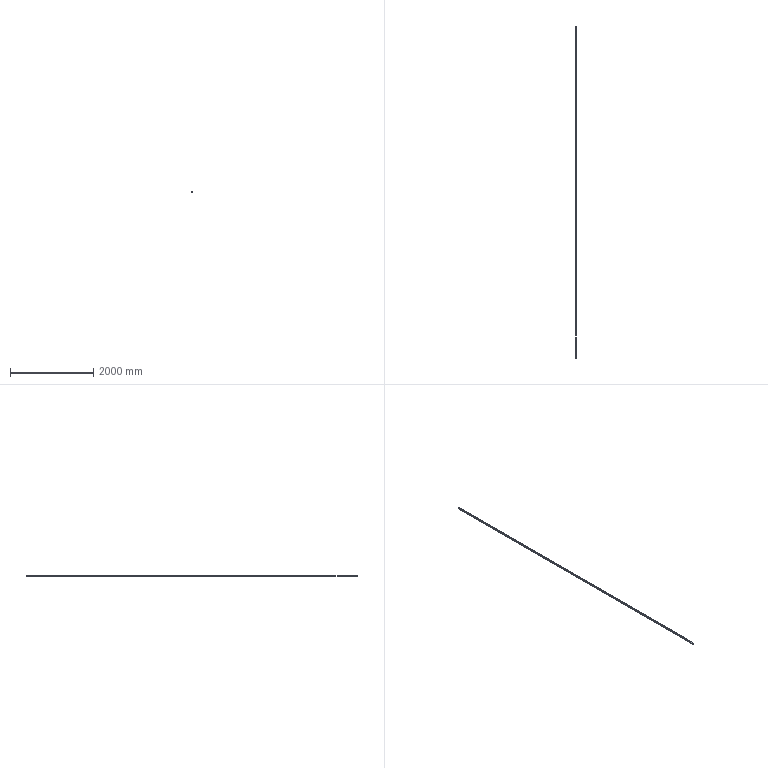Component | SolidWorks | MirrorFence3-10_Mirror30X30X3-7440-1 | 3 solids | 54 faces | volume 2380455 mm3 | plane 30 | cylinder 24 | commonest cylinder face diameters 12 x12 6 x12